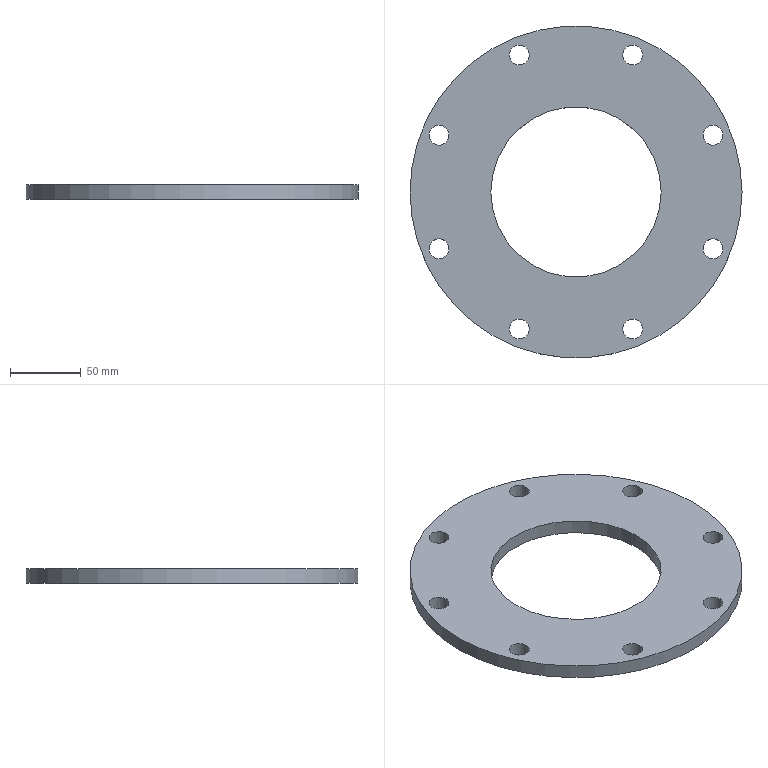Component | NX | CH3404-1 | 1 solid | 16 faces | volume 294430 mm3 | cylinder 12 | plane 4 | commonest cylinder face diameters 14 x8 234 x1 120 x1 161 x1 150 x1